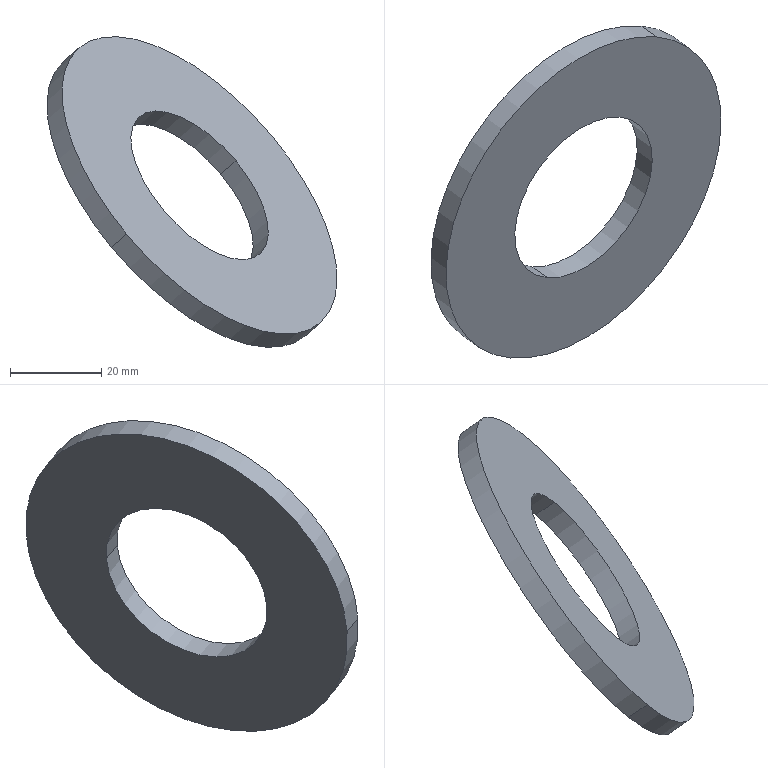Component | SolidWorks | Bolt40x20x5-1 | 1 solid | 6 faces | box 63.45 x 72.72 x 67.97 mm | volume 18850 mm3 | cylinder 4 | plane 2 | commonest cylinder face diameters 40 x2 80 x2 | material Copper
build123d program:
from build123d import *

# Parameters (mm, degrees)
SKETCH1_R           = 40
SKETCH1_R_2         = 20
BOSS_EXTRUDE1_DEPTH = 5


with BuildPart() as part:
    # Sketch1 → Boss-Extrude1 (new body)
    with BuildSketch(Plane(origin=(0, 0, 0), x_dir=(1, 0, 0), z_dir=(0, 1, 0))):
        with Locations(Location((0, 0, 0), (0, 0, 270))):
            Circle(SKETCH1_R)
        with Locations(Location((0, 0, 0), (0, 0, 270))):
            Circle(SKETCH1_R_2, mode=Mode.SUBTRACT)
    extrude(amount=BOSS_EXTRUDE1_DEPTH)


solid = part.part

# Placed as in the assembly
solid = solid.moved(Location((-297.64, -1560.03, 10.595), (-9.823, -36.737, -124.654)))
STEP:
#1=COLOUR_RGB('',0.7922,0.8196,0.9333);
#2=FILL_AREA_STYLE_COLOUR('',#1);
#3=FILL_AREA_STYLE('',(#2));
#4=SURFACE_STYLE_FILL_AREA(#3);
#5=SURFACE_SIDE_STYLE('',(#4));
#6=SURFACE_STYLE_USAGE(.BOTH.,#5);
#7=PRESENTATION_STYLE_ASSIGNMENT((#6));
#8=CARTESIAN_POINT('',(-11.404,-60.728,0.627));
#9=VERTEX_POINT('',#8);
#10=CARTESIAN_POINT('',(-12.032,-62.109,0.2073));
#11=VERTEX_POINT('',#10);
#12=CARTESIAN_POINT('',(-11.718,-61.419,0.4171));
#13=DIRECTION('',(-0.6592,0.4763,-0.5818));
#14=DIRECTION('',(-0.3988,-0.8775,-0.2665));
#15=AXIS2_PLACEMENT_3D('',#12,#13,#14);
#16=CIRCLE('',#15,0.7874);
#17=EDGE_CURVE('',#9,#11,#16,.T.);
#18=ORIENTED_EDGE('',*,*,#17,.T.);
#19=CARTESIAN_POINT('',(-11.902,-62.203,0.3218));
#20=VERTEX_POINT('',#19);
#21=CARTESIAN_POINT('',(-12.032,-62.109,0.2073));
#22=DIRECTION('',(0.6592,-0.4763,0.5818));
#23=VECTOR('',#22,39.37);
#24=LINE('',#21,#23);
#25=EDGE_CURVE('',#11,#20,#24,.T.);
#26=ORIENTED_EDGE('',*,*,#25,.T.);
#27=CARTESIAN_POINT('',(-11.274,-60.821,0.7415));
#28=VERTEX_POINT('',#27);
#29=CARTESIAN_POINT('',(-11.588,-61.512,0.5317));
#30=DIRECTION('',(-0.6592,0.4763,-0.5818));
#31=DIRECTION('',(-0.3988,-0.8775,-0.2665));
#32=AXIS2_PLACEMENT_3D('',#29,#30,#31);
#33=CIRCLE('',#32,0.7874);
#34=EDGE_CURVE('',#28,#20,#33,.T.);
#35=ORIENTED_EDGE('',*,*,#34,.F.);
#36=CARTESIAN_POINT('',(-11.404,-60.728,0.627));
#37=DIRECTION('',(0.6592,-0.4763,0.5818));
#38=VECTOR('',#37,39.37);
#39=LINE('',#36,#38);
#40=EDGE_CURVE('',#9,#28,#39,.T.);
#41=ORIENTED_EDGE('',*,*,#40,.F.);
#42=EDGE_LOOP('',(#18,#26,#35,#41));
#43=FACE_OUTER_BOUND('',#42,.T.);
#44=CARTESIAN_POINT('',(-11.718,-61.419,0.4171));
#45=DIRECTION('',(0.6592,-0.4763,0.5818));
#46=DIRECTION('',(0.3988,0.8775,0.2665));
#47=AXIS2_PLACEMENT_3D('',#44,#45,#46);
#48=CYLINDRICAL_SURFACE('',#47,0.7874);
#49=ADVANCED_FACE('',(#43),#48,.F.);
#50=CARTESIAN_POINT('',(-12.346,-62.8,-0.00255));
#51=VERTEX_POINT('',#50);
#52=CARTESIAN_POINT('',(-11.09,-60.037,0.8368));
#53=VERTEX_POINT('',#52);
#54=CARTESIAN_POINT('',(-11.718,-61.419,0.4171));
#55=DIRECTION('',(-0.6592,0.4763,-0.5818));
#56=DIRECTION('',(-0.3988,-0.8775,-0.2665));
#57=AXIS2_PLACEMENT_3D('',#54,#55,#56);
#58=CIRCLE('',#57,1.575);
#59=EDGE_CURVE('',#51,#53,#58,.T.);
#60=ORIENTED_EDGE('',*,*,#59,.F.);
#61=CARTESIAN_POINT('',(-12.216,-62.894,0.112));
#62=VERTEX_POINT('',#61);
#63=CARTESIAN_POINT('',(-12.346,-62.8,-0.00255));
#64=DIRECTION('',(0.6592,-0.4763,0.5818));
#65=VECTOR('',#64,39.37);
#66=LINE('',#63,#65);
#67=EDGE_CURVE('',#51,#62,#66,.T.);
#68=ORIENTED_EDGE('',*,*,#67,.T.);
#69=CARTESIAN_POINT('',(-10.96,-60.13,0.9514));
#70=VERTEX_POINT('',#69);
#71=CARTESIAN_POINT('',(-11.588,-61.512,0.5317));
#72=DIRECTION('',(-0.6592,0.4763,-0.5818));
#73=DIRECTION('',(-0.3988,-0.8775,-0.2665));
#74=AXIS2_PLACEMENT_3D('',#71,#72,#73);
#75=CIRCLE('',#74,1.575);
#76=EDGE_CURVE('',#62,#70,#75,.T.);
#77=ORIENTED_EDGE('',*,*,#76,.T.);
#78=CARTESIAN_POINT('',(-11.09,-60.037,0.8368));
#79=DIRECTION('',(0.6592,-0.4763,0.5818));
#80=VECTOR('',#79,39.37);
#81=LINE('',#78,#80);
#82=EDGE_CURVE('',#53,#70,#81,.T.);
#83=ORIENTED_EDGE('',*,*,#82,.F.);
#84=EDGE_LOOP('',(#60,#68,#77,#83));
#85=FACE_OUTER_BOUND('',#84,.T.);
#86=CARTESIAN_POINT('',(-11.718,-61.419,0.4171));
#87=DIRECTION('',(0.6592,-0.4763,0.5818));
#88=DIRECTION('',(0.3988,0.8775,0.2665));
#89=AXIS2_PLACEMENT_3D('',#86,#87,#88);
#90=CYLINDRICAL_SURFACE('',#89,1.575);
#91=ADVANCED_FACE('',(#85),#90,.T.);
#92=CARTESIAN_POINT('',(-11.718,-61.419,0.4171));
#93=DIRECTION('',(-0.6592,0.4763,-0.5818));
#94=DIRECTION('',(-0.3988,-0.8775,-0.2665));
#95=AXIS2_PLACEMENT_3D('',#92,#93,#94);
#96=CIRCLE('',#95,1.575);
#97=EDGE_CURVE('',#53,#51,#96,.T.);
#98=ORIENTED_EDGE('',*,*,#97,.T.);
#99=ORIENTED_EDGE('',*,*,#59,.T.);
#100=EDGE_LOOP('',(#98,#99));
#101=FACE_OUTER_BOUND('',#100,.T.);
#102=ORIENTED_EDGE('',*,*,#17,.F.);
#103=CARTESIAN_POINT('',(-11.718,-61.419,0.4171));
#104=DIRECTION('',(-0.6592,0.4763,-0.5818));
#105=DIRECTION('',(-0.3988,-0.8775,-0.2665));
#106=AXIS2_PLACEMENT_3D('',#103,#104,#105);
#107=CIRCLE('',#106,0.7874);
#108=EDGE_CURVE('',#11,#9,#107,.T.);
#109=ORIENTED_EDGE('',*,*,#108,.F.);
#110=EDGE_LOOP('',(#102,#109));
#111=FACE_BOUND('',#110,.T.);
#112=CARTESIAN_POINT('',(-11.718,-61.419,0.4171));
#113=DIRECTION('',(-0.6592,0.4763,-0.5818));
#114=DIRECTION('',(-0.3988,-0.8775,-0.2665));
#115=AXIS2_PLACEMENT_3D('',#112,#113,#114);
#116=PLANE('',#115);
#117=ADVANCED_FACE('',(#101,#111),#116,.T.);
#118=CARTESIAN_POINT('',(-11.588,-61.512,0.5317));
#119=DIRECTION('',(-0.6592,0.4763,-0.5818));
#120=DIRECTION('',(-0.3988,-0.8775,-0.2665));
#121=AXIS2_PLACEMENT_3D('',#118,#119,#120);
#122=CIRCLE('',#121,1.575);
#123=EDGE_CURVE('',#70,#62,#122,.T.);
#124=ORIENTED_EDGE('',*,*,#123,.F.);
#125=ORIENTED_EDGE('',*,*,#76,.F.);
#126=EDGE_LOOP('',(#124,#125));
#127=FACE_OUTER_BOUND('',#126,.T.);
#128=ORIENTED_EDGE('',*,*,#34,.T.);
#129=CARTESIAN_POINT('',(-11.588,-61.512,0.5317));
#130=DIRECTION('',(-0.6592,0.4763,-0.5818));
#131=DIRECTION('',(-0.3988,-0.8775,-0.2665));
#132=AXIS2_PLACEMENT_3D('',#129,#130,#131);
#133=CIRCLE('',#132,0.7874);
#134=EDGE_CURVE('',#20,#28,#133,.T.);
#135=ORIENTED_EDGE('',*,*,#134,.T.);
#136=EDGE_LOOP('',(#128,#135));
#137=FACE_BOUND('',#136,.T.);
#138=CARTESIAN_POINT('',(-11.588,-61.512,0.5317));
#139=DIRECTION('',(-0.6592,0.4763,-0.5818));
#140=DIRECTION('',(-0.3988,-0.8775,-0.2665));
#141=AXIS2_PLACEMENT_3D('',#138,#139,#140);
#142=PLANE('',#141);
#143=ADVANCED_FACE('',(#127,#137),#142,.F.);
#144=ORIENTED_EDGE('',*,*,#67,.F.);
#145=ORIENTED_EDGE('',*,*,#97,.F.);
#146=ORIENTED_EDGE('',*,*,#82,.T.);
#147=ORIENTED_EDGE('',*,*,#123,.T.);
#148=EDGE_LOOP('',(#144,#145,#146,#147));
#149=FACE_OUTER_BOUND('',#148,.T.);
#150=CARTESIAN_POINT('',(-11.718,-61.419,0.4171));
#151=DIRECTION('',(0.6592,-0.4763,0.5818));
#152=DIRECTION('',(0.3988,0.8775,0.2665));
#153=AXIS2_PLACEMENT_3D('',#150,#151,#152);
#154=CYLINDRICAL_SURFACE('',#153,1.575);
#155=ADVANCED_FACE('',(#149),#154,.T.);
#156=ORIENTED_EDGE('',*,*,#25,.F.);
#157=ORIENTED_EDGE('',*,*,#108,.T.);
#158=ORIENTED_EDGE('',*,*,#40,.T.);
#159=ORIENTED_EDGE('',*,*,#134,.F.);
#160=EDGE_LOOP('',(#156,#157,#158,#159));
#161=FACE_OUTER_BOUND('',#160,.T.);
#162=CARTESIAN_POINT('',(-11.718,-61.419,0.4171));
#163=DIRECTION('',(0.6592,-0.4763,0.5818));
#164=DIRECTION('',(0.3988,0.8775,0.2665));
#165=AXIS2_PLACEMENT_3D('',#162,#163,#164);
#166=CYLINDRICAL_SURFACE('',#165,0.7874);
#167=ADVANCED_FACE('',(#161),#166,.F.);
#168=CLOSED_SHELL('',(#49,#91,#117,#143,#155,#167));
#169=MANIFOLD_SOLID_BREP('',#168);
#170=STYLED_ITEM('',(#7),#169);
#171=(LENGTH_UNIT()NAMED_UNIT(*)SI_UNIT($,.METRE.));
#172=LENGTH_MEASURE_WITH_UNIT(LENGTH_MEASURE(0.0254),#171);
#173=DIMENSIONAL_EXPONENTS(1.,0.,0.,0.,0.,0.,0.);
#174=(CONVERSION_BASED_UNIT('',#172)LENGTH_UNIT()NAMED_UNIT(#173));
#175=UNCERTAINTY_MEASURE_WITH_UNIT(LENGTH_MEASURE(0.00001),#174,'','');
#176=(NAMED_UNIT(*)PLANE_ANGLE_UNIT()SI_UNIT($,.RADIAN.));
#177=(NAMED_UNIT(*)SI_UNIT($,.STERADIAN.)SOLID_ANGLE_UNIT());
#178=(GEOMETRIC_REPRESENTATION_CONTEXT(3)GLOBAL_UNCERTAINTY_ASSIGNED_CONTEXT((#175))GLOBAL_UNIT_ASSIGNED_CONTEXT((#174,#176,#177))REPRESENTATION_CONTEXT('',''));
#179=MECHANICAL_DESIGN_GEOMETRIC_PRESENTATION_REPRESENTATION('',(#170),#178);
#180=PRESENTATION_LAYER_ASSIGNMENT('','',(#170));
#181=CARTESIAN_POINT('',(0.,0.,0.));
#182=DIRECTION('',(0.,0.,1.));
#183=DIRECTION('',(1.,0.,0.));
#184=AXIS2_PLACEMENT_3D('',#181,#182,#183);
#185=(LENGTH_UNIT()NAMED_UNIT(*)SI_UNIT($,.METRE.));
#186=LENGTH_MEASURE_WITH_UNIT(LENGTH_MEASURE(0.0254),#185);
#187=DIMENSIONAL_EXPONENTS(1.,0.,0.,0.,0.,0.,0.);
#188=(CONVERSION_BASED_UNIT('',#186)LENGTH_UNIT()NAMED_UNIT(#187));
#189=UNCERTAINTY_MEASURE_WITH_UNIT(LENGTH_MEASURE(0.00001),#188,'','');
#190=(NAMED_UNIT(*)PLANE_ANGLE_UNIT()SI_UNIT($,.RADIAN.));
#191=(NAMED_UNIT(*)SI_UNIT($,.STERADIAN.)SOLID_ANGLE_UNIT());
#192=(GEOMETRIC_REPRESENTATION_CONTEXT(3)GLOBAL_UNCERTAINTY_ASSIGNED_CONTEXT((#189))GLOBAL_UNIT_ASSIGNED_CONTEXT((#188,#190,#191))REPRESENTATION_CONTEXT('',''));
#193=ADVANCED_BREP_SHAPE_REPRESENTATION('',(#169,#184),#192);